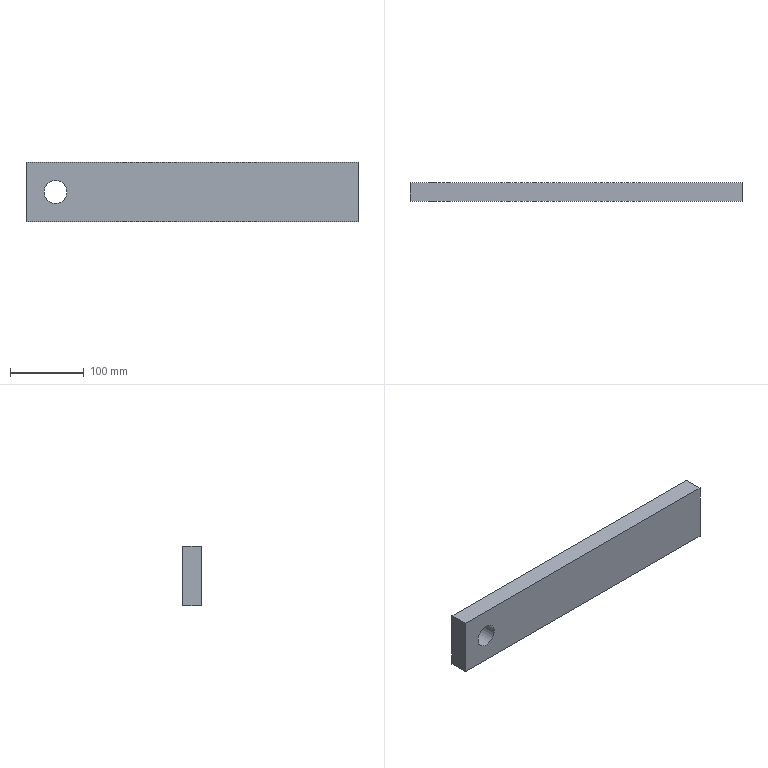Component | NX | CHAPA_GARFO_2 | 1 solid | 7 faces | box 450 x 25.4 x 80 mm | volume 895229 mm3 | plane 6 | cylinder 1 | commonest cylinder face diameters 31 x1
STEP:
#1=CARTESIAN_POINT('',(0.,0.,0.));
#2=DIRECTION('',(0.,0.,1.));
#3=DIRECTION('',(1.,0.,0.));
#4=AXIS2_PLACEMENT_3D('',#1,#2,#3);
#5=CARTESIAN_POINT('',(100.,-672.2,80.));
#6=VERTEX_POINT('',#5);
#7=CARTESIAN_POINT('',(100.,-672.2,-0.));
#8=VERTEX_POINT('',#7);
#9=CARTESIAN_POINT('',(100.,-672.2,80.));
#10=DIRECTION('',(-0.,0.,-1.));
#11=VECTOR('',#10,1.);
#12=LINE('',#9,#11);
#13=CARTESIAN_POINT('',(100.,-646.8,80.));
#14=DIRECTION('',(-1.,0.,0.));
#15=DIRECTION('',(-0.,0.,-1.));
#16=AXIS2_PLACEMENT_3D('',#13,#14,#15);
#17=PLANE('',#16);
#18=CARTESIAN_POINT('',(0.,25.4));
#19=DIRECTION('',(1.,0.));
#20=VECTOR('',#19,1.);
#21=LINE('',#18,#20);
#22=(GEOMETRIC_REPRESENTATION_CONTEXT(2)PARAMETRIC_REPRESENTATION_CONTEXT()REPRESENTATION_CONTEXT('',''));
#23=DEFINITIONAL_REPRESENTATION('',(#21),#22);
#24=PCURVE('',#17,#23);
#25=CARTESIAN_POINT('',(-310.,-672.2,40.));
#26=DIRECTION('',(0.,1.,0.));
#27=DIRECTION('',(0.,0.,-1.));
#28=AXIS2_PLACEMENT_3D('',#25,#26,#27);
#29=PLANE('',#28);
#30=CARTESIAN_POINT('',(-40.,-410.));
#31=DIRECTION('',(1.,0.));
#32=VECTOR('',#31,1.);
#33=LINE('',#30,#32);
#34=(GEOMETRIC_REPRESENTATION_CONTEXT(2)PARAMETRIC_REPRESENTATION_CONTEXT()REPRESENTATION_CONTEXT('',''));
#35=DEFINITIONAL_REPRESENTATION('',(#33),#34);
#36=PCURVE('',#29,#35);
#37=SURFACE_CURVE('',#12,(#24,#36),.PCURVE_S1.);
#38=EDGE_CURVE('',#6,#8,#37,.T.);
#39=ORIENTED_EDGE('',*,*,#38,.T.);
#40=CARTESIAN_POINT('',(100.,-646.8,-0.));
#41=VERTEX_POINT('',#40);
#42=CARTESIAN_POINT('',(100.,-646.8,-0.));
#43=DIRECTION('',(0.,-1.,0.));
#44=VECTOR('',#43,1.);
#45=LINE('',#42,#44);
#46=CARTESIAN_POINT('',(80.,0.));
#47=DIRECTION('',(0.,1.));
#48=VECTOR('',#47,1.);
#49=LINE('',#46,#48);
#50=(GEOMETRIC_REPRESENTATION_CONTEXT(2)PARAMETRIC_REPRESENTATION_CONTEXT()REPRESENTATION_CONTEXT('',''));
#51=DEFINITIONAL_REPRESENTATION('',(#49),#50);
#52=PCURVE('',#17,#51);
#53=CARTESIAN_POINT('',(100.,-646.8,-0.));
#54=DIRECTION('',(0.,0.,1.));
#55=DIRECTION('',(-1.,0.,0.));
#56=AXIS2_PLACEMENT_3D('',#53,#54,#55);
#57=PLANE('',#56);
#58=CARTESIAN_POINT('',(0.,0.));
#59=DIRECTION('',(0.,1.));
#60=VECTOR('',#59,1.);
#61=LINE('',#58,#60);
#62=(GEOMETRIC_REPRESENTATION_CONTEXT(2)PARAMETRIC_REPRESENTATION_CONTEXT()REPRESENTATION_CONTEXT('',''));
#63=DEFINITIONAL_REPRESENTATION('',(#61),#62);
#64=PCURVE('',#57,#63);
#65=SURFACE_CURVE('',#45,(#52,#64),.PCURVE_S1.);
#66=EDGE_CURVE('',#41,#8,#65,.T.);
#67=ORIENTED_EDGE('',*,*,#66,.F.);
#68=CARTESIAN_POINT('',(100.,-646.8,80.));
#69=VERTEX_POINT('',#68);
#70=CARTESIAN_POINT('',(100.,-646.8,80.));
#71=DIRECTION('',(-0.,0.,-1.));
#72=VECTOR('',#71,1.);
#73=LINE('',#70,#72);
#74=CARTESIAN_POINT('',(0.,0.));
#75=DIRECTION('',(1.,0.));
#76=VECTOR('',#75,1.);
#77=LINE('',#74,#76);
#78=(GEOMETRIC_REPRESENTATION_CONTEXT(2)PARAMETRIC_REPRESENTATION_CONTEXT()REPRESENTATION_CONTEXT('',''));
#79=DEFINITIONAL_REPRESENTATION('',(#77),#78);
#80=PCURVE('',#17,#79);
#81=CARTESIAN_POINT('',(-310.,-646.8,40.));
#82=DIRECTION('',(0.,1.,0.));
#83=DIRECTION('',(0.,0.,-1.));
#84=AXIS2_PLACEMENT_3D('',#81,#82,#83);
#85=PLANE('',#84);
#86=CARTESIAN_POINT('',(-40.,-410.));
#87=DIRECTION('',(1.,0.));
#88=VECTOR('',#87,1.);
#89=LINE('',#86,#88);
#90=(GEOMETRIC_REPRESENTATION_CONTEXT(2)PARAMETRIC_REPRESENTATION_CONTEXT()REPRESENTATION_CONTEXT('',''));
#91=DEFINITIONAL_REPRESENTATION('',(#89),#90);
#92=PCURVE('',#85,#91);
#93=SURFACE_CURVE('',#73,(#80,#92),.PCURVE_S1.);
#94=EDGE_CURVE('',#69,#41,#93,.T.);
#95=ORIENTED_EDGE('',*,*,#94,.F.);
#96=CARTESIAN_POINT('',(100.,-646.8,80.));
#97=DIRECTION('',(0.,-1.,0.));
#98=VECTOR('',#97,1.);
#99=LINE('',#96,#98);
#100=CARTESIAN_POINT('',(0.,0.));
#101=DIRECTION('',(0.,1.));
#102=VECTOR('',#101,1.);
#103=LINE('',#100,#102);
#104=(GEOMETRIC_REPRESENTATION_CONTEXT(2)PARAMETRIC_REPRESENTATION_CONTEXT()REPRESENTATION_CONTEXT('',''));
#105=DEFINITIONAL_REPRESENTATION('',(#103),#104);
#106=PCURVE('',#17,#105);
#107=CARTESIAN_POINT('',(-350.,-646.8,80.));
#108=DIRECTION('',(-0.,0.,-1.));
#109=DIRECTION('',(1.,0.,-0.));
#110=AXIS2_PLACEMENT_3D('',#107,#108,#109);
#111=PLANE('',#110);
#112=CARTESIAN_POINT('',(450.,0.));
#113=DIRECTION('',(0.,1.));
#114=VECTOR('',#113,1.);
#115=LINE('',#112,#114);
#116=(GEOMETRIC_REPRESENTATION_CONTEXT(2)PARAMETRIC_REPRESENTATION_CONTEXT()REPRESENTATION_CONTEXT('',''));
#117=DEFINITIONAL_REPRESENTATION('',(#115),#116);
#118=PCURVE('',#111,#117);
#119=SURFACE_CURVE('',#99,(#106,#118),.PCURVE_S1.);
#120=EDGE_CURVE('',#69,#6,#119,.T.);
#121=ORIENTED_EDGE('',*,*,#120,.T.);
#122=EDGE_LOOP('',(#39,#67,#95,#121));
#123=FACE_BOUND('',#122,.T.);
#124=ADVANCED_FACE('',(#123),#17,.F.);
#125=CARTESIAN_POINT('',(-350.,-672.2,0.));
#126=VERTEX_POINT('',#125);
#127=CARTESIAN_POINT('',(100.,-672.2,-0.));
#128=DIRECTION('',(-1.,0.,0.));
#129=VECTOR('',#128,1.);
#130=LINE('',#127,#129);
#131=CARTESIAN_POINT('',(0.,25.4));
#132=DIRECTION('',(1.,0.));
#133=VECTOR('',#132,1.);
#134=LINE('',#131,#133);
#135=(GEOMETRIC_REPRESENTATION_CONTEXT(2)PARAMETRIC_REPRESENTATION_CONTEXT()REPRESENTATION_CONTEXT('',''));
#136=DEFINITIONAL_REPRESENTATION('',(#134),#135);
#137=PCURVE('',#57,#136);
#138=CARTESIAN_POINT('',(40.,-410.));
#139=DIRECTION('',(-0.,1.));
#140=VECTOR('',#139,1.);
#141=LINE('',#138,#140);
#142=(GEOMETRIC_REPRESENTATION_CONTEXT(2)PARAMETRIC_REPRESENTATION_CONTEXT()REPRESENTATION_CONTEXT('',''));
#143=DEFINITIONAL_REPRESENTATION('',(#141),#142);
#144=PCURVE('',#29,#143);
#145=SURFACE_CURVE('',#130,(#137,#144),.PCURVE_S1.);
#146=EDGE_CURVE('',#8,#126,#145,.T.);
#147=ORIENTED_EDGE('',*,*,#146,.T.);
#148=CARTESIAN_POINT('',(-350.,-646.8,0.));
#149=VERTEX_POINT('',#148);
#150=CARTESIAN_POINT('',(-350.,-646.8,0.));
#151=DIRECTION('',(0.,-1.,0.));
#152=VECTOR('',#151,1.);
#153=LINE('',#150,#152);
#154=CARTESIAN_POINT('',(450.,0.));
#155=DIRECTION('',(0.,1.));
#156=VECTOR('',#155,1.);
#157=LINE('',#154,#156);
#158=(GEOMETRIC_REPRESENTATION_CONTEXT(2)PARAMETRIC_REPRESENTATION_CONTEXT()REPRESENTATION_CONTEXT('',''));
#159=DEFINITIONAL_REPRESENTATION('',(#157),#158);
#160=PCURVE('',#57,#159);
#161=CARTESIAN_POINT('',(-350.,-646.8,0.));
#162=DIRECTION('',(1.,0.,0.));
#163=DIRECTION('',(0.,0.,1.));
#164=AXIS2_PLACEMENT_3D('',#161,#162,#163);
#165=PLANE('',#164);
#166=CARTESIAN_POINT('',(0.,0.));
#167=DIRECTION('',(0.,1.));
#168=VECTOR('',#167,1.);
#169=LINE('',#166,#168);
#170=(GEOMETRIC_REPRESENTATION_CONTEXT(2)PARAMETRIC_REPRESENTATION_CONTEXT()REPRESENTATION_CONTEXT('',''));
#171=DEFINITIONAL_REPRESENTATION('',(#169),#170);
#172=PCURVE('',#165,#171);
#173=SURFACE_CURVE('',#153,(#160,#172),.PCURVE_S1.);
#174=EDGE_CURVE('',#149,#126,#173,.T.);
#175=ORIENTED_EDGE('',*,*,#174,.F.);
#176=CARTESIAN_POINT('',(100.,-646.8,-0.));
#177=DIRECTION('',(-1.,0.,0.));
#178=VECTOR('',#177,1.);
#179=LINE('',#176,#178);
#180=CARTESIAN_POINT('',(0.,0.));
#181=DIRECTION('',(1.,0.));
#182=VECTOR('',#181,1.);
#183=LINE('',#180,#182);
#184=(GEOMETRIC_REPRESENTATION_CONTEXT(2)PARAMETRIC_REPRESENTATION_CONTEXT()REPRESENTATION_CONTEXT('',''));
#185=DEFINITIONAL_REPRESENTATION('',(#183),#184);
#186=PCURVE('',#57,#185);
#187=CARTESIAN_POINT('',(40.,-410.));
#188=DIRECTION('',(-0.,1.));
#189=VECTOR('',#188,1.);
#190=LINE('',#187,#189);
#191=(GEOMETRIC_REPRESENTATION_CONTEXT(2)PARAMETRIC_REPRESENTATION_CONTEXT()REPRESENTATION_CONTEXT('',''));
#192=DEFINITIONAL_REPRESENTATION('',(#190),#191);
#193=PCURVE('',#85,#192);
#194=SURFACE_CURVE('',#179,(#186,#193),.PCURVE_S1.);
#195=EDGE_CURVE('',#41,#149,#194,.T.);
#196=ORIENTED_EDGE('',*,*,#195,.F.);
#197=ORIENTED_EDGE('',*,*,#66,.T.);
#198=EDGE_LOOP('',(#147,#175,#196,#197));
#199=FACE_BOUND('',#198,.T.);
#200=ADVANCED_FACE('',(#199),#57,.F.);
#201=CARTESIAN_POINT('',(-350.,-672.2,80.));
#202=VERTEX_POINT('',#201);
#203=CARTESIAN_POINT('',(-350.,-672.2,0.));
#204=DIRECTION('',(0.,0.,1.));
#205=VECTOR('',#204,1.);
#206=LINE('',#203,#205);
#207=CARTESIAN_POINT('',(0.,25.4));
#208=DIRECTION('',(1.,0.));
#209=VECTOR('',#208,1.);
#210=LINE('',#207,#209);
#211=(GEOMETRIC_REPRESENTATION_CONTEXT(2)PARAMETRIC_REPRESENTATION_CONTEXT()REPRESENTATION_CONTEXT('',''));
#212=DEFINITIONAL_REPRESENTATION('',(#210),#211);
#213=PCURVE('',#165,#212);
#214=CARTESIAN_POINT('',(40.,40.));
#215=DIRECTION('',(-1.,0.));
#216=VECTOR('',#215,1.);
#217=LINE('',#214,#216);
#218=(GEOMETRIC_REPRESENTATION_CONTEXT(2)PARAMETRIC_REPRESENTATION_CONTEXT()REPRESENTATION_CONTEXT('',''));
#219=DEFINITIONAL_REPRESENTATION('',(#217),#218);
#220=PCURVE('',#29,#219);
#221=SURFACE_CURVE('',#206,(#213,#220),.PCURVE_S1.);
#222=EDGE_CURVE('',#126,#202,#221,.T.);
#223=ORIENTED_EDGE('',*,*,#222,.T.);
#224=CARTESIAN_POINT('',(-350.,-646.8,80.));
#225=VERTEX_POINT('',#224);
#226=CARTESIAN_POINT('',(-350.,-646.8,80.));
#227=DIRECTION('',(0.,-1.,0.));
#228=VECTOR('',#227,1.);
#229=LINE('',#226,#228);
#230=CARTESIAN_POINT('',(80.,0.));
#231=DIRECTION('',(0.,1.));
#232=VECTOR('',#231,1.);
#233=LINE('',#230,#232);
#234=(GEOMETRIC_REPRESENTATION_CONTEXT(2)PARAMETRIC_REPRESENTATION_CONTEXT()REPRESENTATION_CONTEXT('',''));
#235=DEFINITIONAL_REPRESENTATION('',(#233),#234);
#236=PCURVE('',#165,#235);
#237=CARTESIAN_POINT('',(0.,0.));
#238=DIRECTION('',(0.,1.));
#239=VECTOR('',#238,1.);
#240=LINE('',#237,#239);
#241=(GEOMETRIC_REPRESENTATION_CONTEXT(2)PARAMETRIC_REPRESENTATION_CONTEXT()REPRESENTATION_CONTEXT('',''));
#242=DEFINITIONAL_REPRESENTATION('',(#240),#241);
#243=PCURVE('',#111,#242);
#244=SURFACE_CURVE('',#229,(#236,#243),.PCURVE_S1.);
#245=EDGE_CURVE('',#225,#202,#244,.T.);
#246=ORIENTED_EDGE('',*,*,#245,.F.);
#247=CARTESIAN_POINT('',(-350.,-646.8,0.));
#248=DIRECTION('',(0.,0.,1.));
#249=VECTOR('',#248,1.);
#250=LINE('',#247,#249);
#251=CARTESIAN_POINT('',(0.,0.));
#252=DIRECTION('',(1.,0.));
#253=VECTOR('',#252,1.);
#254=LINE('',#251,#253);
#255=(GEOMETRIC_REPRESENTATION_CONTEXT(2)PARAMETRIC_REPRESENTATION_CONTEXT()REPRESENTATION_CONTEXT('',''));
#256=DEFINITIONAL_REPRESENTATION('',(#254),#255);
#257=PCURVE('',#165,#256);
#258=CARTESIAN_POINT('',(40.,40.));
#259=DIRECTION('',(-1.,0.));
#260=VECTOR('',#259,1.);
#261=LINE('',#258,#260);
#262=(GEOMETRIC_REPRESENTATION_CONTEXT(2)PARAMETRIC_REPRESENTATION_CONTEXT()REPRESENTATION_CONTEXT('',''));
#263=DEFINITIONAL_REPRESENTATION('',(#261),#262);
#264=PCURVE('',#85,#263);
#265=SURFACE_CURVE('',#250,(#257,#264),.PCURVE_S1.);
#266=EDGE_CURVE('',#149,#225,#265,.T.);
#267=ORIENTED_EDGE('',*,*,#266,.F.);
#268=ORIENTED_EDGE('',*,*,#174,.T.);
#269=EDGE_LOOP('',(#223,#246,#267,#268));
#270=FACE_BOUND('',#269,.T.);
#271=ADVANCED_FACE('',(#270),#165,.F.);
#272=CARTESIAN_POINT('',(-350.,-672.2,80.));
#273=DIRECTION('',(1.,0.,-0.));
#274=VECTOR('',#273,1.);
#275=LINE('',#272,#274);
#276=CARTESIAN_POINT('',(0.,25.4));
#277=DIRECTION('',(1.,0.));
#278=VECTOR('',#277,1.);
#279=LINE('',#276,#278);
#280=(GEOMETRIC_REPRESENTATION_CONTEXT(2)PARAMETRIC_REPRESENTATION_CONTEXT()REPRESENTATION_CONTEXT('',''));
#281=DEFINITIONAL_REPRESENTATION('',(#279),#280);
#282=PCURVE('',#111,#281);
#283=CARTESIAN_POINT('',(-40.,40.));
#284=DIRECTION('',(0.,-1.));
#285=VECTOR('',#284,1.);
#286=LINE('',#283,#285);
#287=(GEOMETRIC_REPRESENTATION_CONTEXT(2)PARAMETRIC_REPRESENTATION_CONTEXT()REPRESENTATION_CONTEXT('',''));
#288=DEFINITIONAL_REPRESENTATION('',(#286),#287);
#289=PCURVE('',#29,#288);
#290=SURFACE_CURVE('',#275,(#282,#289),.PCURVE_S1.);
#291=EDGE_CURVE('',#202,#6,#290,.T.);
#292=ORIENTED_EDGE('',*,*,#291,.T.);
#293=ORIENTED_EDGE('',*,*,#120,.F.);
#294=CARTESIAN_POINT('',(-350.,-646.8,80.));
#295=DIRECTION('',(1.,0.,-0.));
#296=VECTOR('',#295,1.);
#297=LINE('',#294,#296);
#298=CARTESIAN_POINT('',(0.,0.));
#299=DIRECTION('',(1.,0.));
#300=VECTOR('',#299,1.);
#301=LINE('',#298,#300);
#302=(GEOMETRIC_REPRESENTATION_CONTEXT(2)PARAMETRIC_REPRESENTATION_CONTEXT()REPRESENTATION_CONTEXT('',''));
#303=DEFINITIONAL_REPRESENTATION('',(#301),#302);
#304=PCURVE('',#111,#303);
#305=CARTESIAN_POINT('',(-40.,40.));
#306=DIRECTION('',(0.,-1.));
#307=VECTOR('',#306,1.);
#308=LINE('',#305,#307);
#309=(GEOMETRIC_REPRESENTATION_CONTEXT(2)PARAMETRIC_REPRESENTATION_CONTEXT()REPRESENTATION_CONTEXT('',''));
#310=DEFINITIONAL_REPRESENTATION('',(#308),#309);
#311=PCURVE('',#85,#310);
#312=SURFACE_CURVE('',#297,(#304,#311),.PCURVE_S1.);
#313=EDGE_CURVE('',#225,#69,#312,.T.);
#314=ORIENTED_EDGE('',*,*,#313,.F.);
#315=ORIENTED_EDGE('',*,*,#245,.T.);
#316=EDGE_LOOP('',(#292,#293,#314,#315));
#317=FACE_BOUND('',#316,.T.);
#318=ADVANCED_FACE('',(#317),#111,.F.);
#319=CARTESIAN_POINT('',(-325.5,-646.8,40.));
#320=VERTEX_POINT('',#319);
#321=CARTESIAN_POINT('',(-310.,-646.8,40.));
#322=DIRECTION('',(0.,1.,0.));
#323=DIRECTION('',(-1.,0.,0.));
#324=AXIS2_PLACEMENT_3D('',#321,#322,#323);
#325=CIRCLE('',#324,15.5);
#326=CARTESIAN_POINT('',(-310.,-646.8,40.));
#327=DIRECTION('',(0.,-1.,0.));
#328=DIRECTION('',(0.,0.,1.));
#329=AXIS2_PLACEMENT_3D('',#326,#327,#328);
#330=CYLINDRICAL_SURFACE('',#329,15.5);
#331=CARTESIAN_POINT('',(7.854,0.));
#332=DIRECTION('',(-1.,0.));
#333=VECTOR('',#332,1.);
#334=LINE('',#331,#333);
#335=(GEOMETRIC_REPRESENTATION_CONTEXT(2)PARAMETRIC_REPRESENTATION_CONTEXT()REPRESENTATION_CONTEXT('',''));
#336=DEFINITIONAL_REPRESENTATION('',(#334),#335);
#337=PCURVE('',#330,#336);
#338=CARTESIAN_POINT('',(0.,0.));
#339=DIRECTION('',(0.,1.));
#340=AXIS2_PLACEMENT_2D('',#338,#339);
#341=CIRCLE('',#340,15.5);
#342=(GEOMETRIC_REPRESENTATION_CONTEXT(2)PARAMETRIC_REPRESENTATION_CONTEXT()REPRESENTATION_CONTEXT('',''));
#343=DEFINITIONAL_REPRESENTATION('',(#341),#342);
#344=PCURVE('',#85,#343);
#345=SURFACE_CURVE('',#325,(#337,#344),.PCURVE_S1.);
#346=EDGE_CURVE('',#320,#320,#345,.T.);
#347=ORIENTED_EDGE('',*,*,#346,.F.);
#348=CARTESIAN_POINT('',(-325.5,-672.2,40.));
#349=VERTEX_POINT('',#348);
#350=CARTESIAN_POINT('',(-325.5,-646.8,40.));
#351=CARTESIAN_POINT('',(-325.5,-672.2,40.));
#352=B_SPLINE_CURVE_WITH_KNOTS('',1,(#350,#351),.UNSPECIFIED.,.F.,.F.,(2,2),(0.,25.4),.PIECEWISE_BEZIER_KNOTS.);
#353=CARTESIAN_POINT('',(7.854,0.));
#354=DIRECTION('',(0.,1.));
#355=VECTOR('',#354,1.);
#356=LINE('',#353,#355);
#357=(GEOMETRIC_REPRESENTATION_CONTEXT(2)PARAMETRIC_REPRESENTATION_CONTEXT()REPRESENTATION_CONTEXT('',''));
#358=DEFINITIONAL_REPRESENTATION('',(#356),#357);
#359=PCURVE('',#330,#358);
#360=CARTESIAN_POINT('',(1.571,0.));
#361=DIRECTION('',(0.,1.));
#362=VECTOR('',#361,1.);
#363=LINE('',#360,#362);
#364=(GEOMETRIC_REPRESENTATION_CONTEXT(2)PARAMETRIC_REPRESENTATION_CONTEXT()REPRESENTATION_CONTEXT('',''));
#365=DEFINITIONAL_REPRESENTATION('',(#363),#364);
#366=PCURVE('',#330,#365);
#367=SEAM_CURVE('',#352,(#359,#366),.PCURVE_S1.);
#368=EDGE_CURVE('',#320,#349,#367,.T.);
#369=ORIENTED_EDGE('',*,*,#368,.T.);
#370=CARTESIAN_POINT('',(-310.,-672.2,40.));
#371=DIRECTION('',(0.,1.,0.));
#372=DIRECTION('',(-1.,0.,0.));
#373=AXIS2_PLACEMENT_3D('',#370,#371,#372);
#374=CIRCLE('',#373,15.5);
#375=CARTESIAN_POINT('',(7.854,25.4));
#376=DIRECTION('',(-1.,0.));
#377=VECTOR('',#376,1.);
#378=LINE('',#375,#377);
#379=(GEOMETRIC_REPRESENTATION_CONTEXT(2)PARAMETRIC_REPRESENTATION_CONTEXT()REPRESENTATION_CONTEXT('',''));
#380=DEFINITIONAL_REPRESENTATION('',(#378),#379);
#381=PCURVE('',#330,#380);
#382=CARTESIAN_POINT('',(0.,0.));
#383=DIRECTION('',(0.,1.));
#384=AXIS2_PLACEMENT_2D('',#382,#383);
#385=CIRCLE('',#384,15.5);
#386=(GEOMETRIC_REPRESENTATION_CONTEXT(2)PARAMETRIC_REPRESENTATION_CONTEXT()REPRESENTATION_CONTEXT('',''));
#387=DEFINITIONAL_REPRESENTATION('',(#385),#386);
#388=PCURVE('',#29,#387);
#389=SURFACE_CURVE('',#374,(#381,#388),.PCURVE_S1.);
#390=EDGE_CURVE('',#349,#349,#389,.T.);
#391=ORIENTED_EDGE('',*,*,#390,.T.);
#392=ORIENTED_EDGE('',*,*,#368,.F.);
#393=EDGE_LOOP('',(#347,#369,#391,#392));
#394=FACE_BOUND('',#393,.F.);
#395=ADVANCED_FACE('',(#394),#330,.F.);
#396=ORIENTED_EDGE('',*,*,#94,.T.);
#397=ORIENTED_EDGE('',*,*,#195,.T.);
#398=ORIENTED_EDGE('',*,*,#266,.T.);
#399=ORIENTED_EDGE('',*,*,#313,.T.);
#400=EDGE_LOOP('',(#396,#397,#398,#399));
#401=FACE_BOUND('',#400,.T.);
#402=ORIENTED_EDGE('',*,*,#346,.F.);
#403=EDGE_LOOP('',(#402));
#404=FACE_BOUND('',#403,.T.);
#405=ADVANCED_FACE('',(#401,#404),#85,.T.);
#406=ORIENTED_EDGE('',*,*,#38,.F.);
#407=ORIENTED_EDGE('',*,*,#291,.F.);
#408=ORIENTED_EDGE('',*,*,#222,.F.);
#409=ORIENTED_EDGE('',*,*,#146,.F.);
#410=EDGE_LOOP('',(#406,#407,#408,#409));
#411=FACE_BOUND('',#410,.T.);
#412=ORIENTED_EDGE('',*,*,#390,.T.);
#413=EDGE_LOOP('',(#412));
#414=FACE_BOUND('',#413,.T.);
#415=ADVANCED_FACE('',(#411,#414),#29,.F.);
#416=CLOSED_SHELL('',(#124,#200,#271,#318,#395,#405,#415));
#417=MANIFOLD_SOLID_BREP('',#416);
#418=(LENGTH_UNIT()NAMED_UNIT(*)SI_UNIT(.MILLI.,.METRE.));
#419=UNCERTAINTY_MEASURE_WITH_UNIT(LENGTH_MEASURE(0.000002),#418,'','');
#420=(NAMED_UNIT(*)PLANE_ANGLE_UNIT()SI_UNIT($,.RADIAN.));
#421=(NAMED_UNIT(*)SI_UNIT($,.STERADIAN.)SOLID_ANGLE_UNIT());
#422=(GEOMETRIC_REPRESENTATION_CONTEXT(3)GLOBAL_UNCERTAINTY_ASSIGNED_CONTEXT((#419))GLOBAL_UNIT_ASSIGNED_CONTEXT((#418,#420,#421))REPRESENTATION_CONTEXT('',''));
#423=ADVANCED_BREP_SHAPE_REPRESENTATION('',(#4,#417),#422);